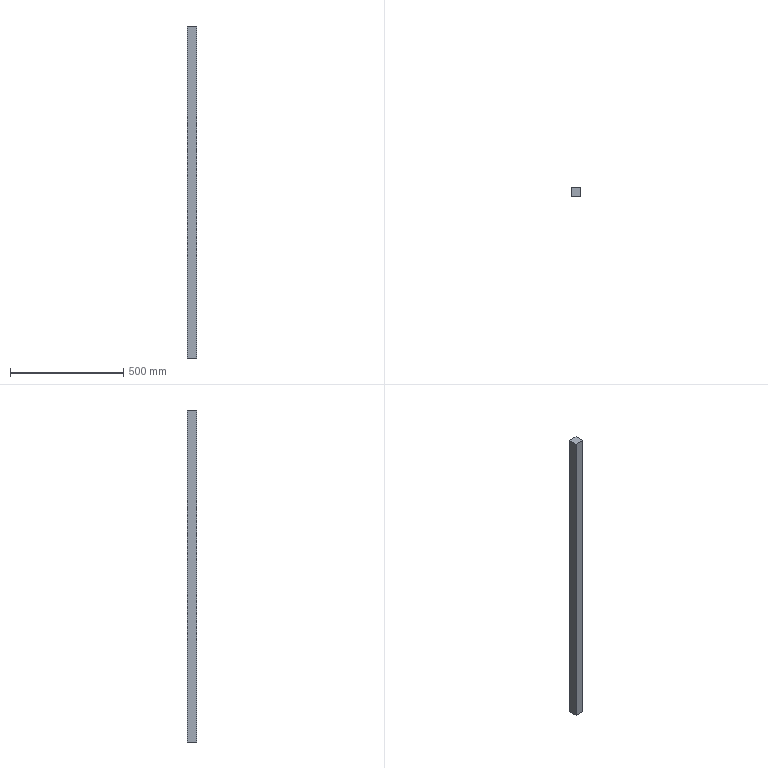Component | SolidWorks | SofaBackrest-1_SupportBar-1 | 1 solid | 6 faces | box 40 x 40 x 1468 mm | volume 2348800 mm3 | plane 6
build123d program:
from build123d import *

# Parameters (mm, degrees)
SKETCH1_W           = 40
SKETCH1_H           = 40
BOSS_EXTRUDE1_DEPTH = 1468


with BuildPart() as part:
    # Sketch1 → Boss-Extrude1 (new body)
    with BuildSketch(Plane.XY):
        with Locations((-12.665, -1.306)):
            Rectangle(SKETCH1_W, SKETCH1_H)
    extrude(amount=BOSS_EXTRUDE1_DEPTH)


solid = part.part

# Placed as in the assembly
solid = solid.moved(Location((310.484, 76.908, 846), (0, 0, 0)))
STEP:
#1=COLOUR_RGB('',0.7922,0.8196,0.9333);
#2=FILL_AREA_STYLE_COLOUR('',#1);
#3=FILL_AREA_STYLE('',(#2));
#4=SURFACE_STYLE_FILL_AREA(#3);
#5=SURFACE_SIDE_STYLE('',(#4));
#6=SURFACE_STYLE_USAGE(.BOTH.,#5);
#7=PRESENTATION_STYLE_ASSIGNMENT((#6));
#8=CARTESIAN_POINT('',(10.938,3.764,33.307));
#9=VERTEX_POINT('',#8);
#10=CARTESIAN_POINT('',(10.938,2.189,33.307));
#11=VERTEX_POINT('',#10);
#12=CARTESIAN_POINT('',(10.938,3.764,33.307));
#13=DIRECTION('',(0.,-1.,0.));
#14=VECTOR('',#13,39.37);
#15=LINE('',#12,#14);
#16=EDGE_CURVE('',#9,#11,#15,.T.);
#17=ORIENTED_EDGE('',*,*,#16,.T.);
#18=CARTESIAN_POINT('',(10.938,2.189,91.102));
#19=VERTEX_POINT('',#18);
#20=CARTESIAN_POINT('',(10.938,2.189,91.102));
#21=DIRECTION('',(0.,0.,-1.));
#22=VECTOR('',#21,39.37);
#23=LINE('',#20,#22);
#24=EDGE_CURVE('',#19,#11,#23,.T.);
#25=ORIENTED_EDGE('',*,*,#24,.F.);
#26=CARTESIAN_POINT('',(10.938,3.764,91.102));
#27=VERTEX_POINT('',#26);
#28=CARTESIAN_POINT('',(10.938,3.764,91.102));
#29=DIRECTION('',(0.,-1.,0.));
#30=VECTOR('',#29,39.37);
#31=LINE('',#28,#30);
#32=EDGE_CURVE('',#27,#19,#31,.T.);
#33=ORIENTED_EDGE('',*,*,#32,.F.);
#34=CARTESIAN_POINT('',(10.938,3.764,91.102));
#35=DIRECTION('',(0.,0.,-1.));
#36=VECTOR('',#35,39.37);
#37=LINE('',#34,#36);
#38=EDGE_CURVE('',#27,#9,#37,.T.);
#39=ORIENTED_EDGE('',*,*,#38,.T.);
#40=EDGE_LOOP('',(#17,#25,#33,#39));
#41=FACE_OUTER_BOUND('',#40,.T.);
#42=CARTESIAN_POINT('',(10.938,3.764,91.102));
#43=DIRECTION('',(1.,0.,0.));
#44=DIRECTION('',(-0.,1.,0.));
#45=AXIS2_PLACEMENT_3D('',#42,#43,#44);
#46=PLANE('',#45);
#47=ADVANCED_FACE('',(#41),#46,.F.);
#48=CARTESIAN_POINT('',(12.513,2.189,33.307));
#49=VERTEX_POINT('',#48);
#50=CARTESIAN_POINT('',(10.938,2.189,33.307));
#51=DIRECTION('',(1.,0.,0.));
#52=VECTOR('',#51,39.37);
#53=LINE('',#50,#52);
#54=EDGE_CURVE('',#11,#49,#53,.T.);
#55=ORIENTED_EDGE('',*,*,#54,.T.);
#56=CARTESIAN_POINT('',(12.513,2.189,91.102));
#57=VERTEX_POINT('',#56);
#58=CARTESIAN_POINT('',(12.513,2.189,91.102));
#59=DIRECTION('',(0.,0.,-1.));
#60=VECTOR('',#59,39.37);
#61=LINE('',#58,#60);
#62=EDGE_CURVE('',#57,#49,#61,.T.);
#63=ORIENTED_EDGE('',*,*,#62,.F.);
#64=CARTESIAN_POINT('',(10.938,2.189,91.102));
#65=DIRECTION('',(1.,0.,0.));
#66=VECTOR('',#65,39.37);
#67=LINE('',#64,#66);
#68=EDGE_CURVE('',#19,#57,#67,.T.);
#69=ORIENTED_EDGE('',*,*,#68,.F.);
#70=ORIENTED_EDGE('',*,*,#24,.T.);
#71=EDGE_LOOP('',(#55,#63,#69,#70));
#72=FACE_OUTER_BOUND('',#71,.T.);
#73=CARTESIAN_POINT('',(10.938,2.189,91.102));
#74=DIRECTION('',(0.,1.,0.));
#75=DIRECTION('',(0.,0.,1.));
#76=AXIS2_PLACEMENT_3D('',#73,#74,#75);
#77=PLANE('',#76);
#78=ADVANCED_FACE('',(#72),#77,.F.);
#79=CARTESIAN_POINT('',(12.513,3.764,33.307));
#80=VERTEX_POINT('',#79);
#81=CARTESIAN_POINT('',(12.513,3.764,33.307));
#82=DIRECTION('',(-0.,1.,0.));
#83=VECTOR('',#82,39.37);
#84=LINE('',#81,#83);
#85=EDGE_CURVE('',#49,#80,#84,.T.);
#86=ORIENTED_EDGE('',*,*,#85,.T.);
#87=CARTESIAN_POINT('',(12.513,3.764,91.102));
#88=VERTEX_POINT('',#87);
#89=CARTESIAN_POINT('',(12.513,3.764,91.102));
#90=DIRECTION('',(0.,0.,-1.));
#91=VECTOR('',#90,39.37);
#92=LINE('',#89,#91);
#93=EDGE_CURVE('',#88,#80,#92,.T.);
#94=ORIENTED_EDGE('',*,*,#93,.F.);
#95=CARTESIAN_POINT('',(12.513,3.764,91.102));
#96=DIRECTION('',(-0.,1.,0.));
#97=VECTOR('',#96,39.37);
#98=LINE('',#95,#97);
#99=EDGE_CURVE('',#57,#88,#98,.T.);
#100=ORIENTED_EDGE('',*,*,#99,.F.);
#101=ORIENTED_EDGE('',*,*,#62,.T.);
#102=EDGE_LOOP('',(#86,#94,#100,#101));
#103=FACE_OUTER_BOUND('',#102,.T.);
#104=CARTESIAN_POINT('',(12.513,3.764,91.102));
#105=DIRECTION('',(-1.,-0.,0.));
#106=DIRECTION('',(0.,-1.,0.));
#107=AXIS2_PLACEMENT_3D('',#104,#105,#106);
#108=PLANE('',#107);
#109=ADVANCED_FACE('',(#103),#108,.F.);
#110=CARTESIAN_POINT('',(10.938,3.764,33.307));
#111=DIRECTION('',(-1.,0.,0.));
#112=VECTOR('',#111,39.37);
#113=LINE('',#110,#112);
#114=EDGE_CURVE('',#80,#9,#113,.T.);
#115=ORIENTED_EDGE('',*,*,#114,.T.);
#116=ORIENTED_EDGE('',*,*,#38,.F.);
#117=CARTESIAN_POINT('',(10.938,3.764,91.102));
#118=DIRECTION('',(-1.,0.,0.));
#119=VECTOR('',#118,39.37);
#120=LINE('',#117,#119);
#121=EDGE_CURVE('',#88,#27,#120,.T.);
#122=ORIENTED_EDGE('',*,*,#121,.F.);
#123=ORIENTED_EDGE('',*,*,#93,.T.);
#124=EDGE_LOOP('',(#115,#116,#122,#123));
#125=FACE_OUTER_BOUND('',#124,.T.);
#126=CARTESIAN_POINT('',(10.938,3.764,91.102));
#127=DIRECTION('',(0.,-1.,0.));
#128=DIRECTION('',(0.,0.,-1.));
#129=AXIS2_PLACEMENT_3D('',#126,#127,#128);
#130=PLANE('',#129);
#131=ADVANCED_FACE('',(#125),#130,.F.);
#132=ORIENTED_EDGE('',*,*,#32,.T.);
#133=ORIENTED_EDGE('',*,*,#68,.T.);
#134=ORIENTED_EDGE('',*,*,#99,.T.);
#135=ORIENTED_EDGE('',*,*,#121,.T.);
#136=EDGE_LOOP('',(#132,#133,#134,#135));
#137=FACE_OUTER_BOUND('',#136,.T.);
#138=CARTESIAN_POINT('',(12.224,3.028,91.102));
#139=DIRECTION('',(0.,0.,1.));
#140=DIRECTION('',(1.,0.,0.));
#141=AXIS2_PLACEMENT_3D('',#138,#139,#140);
#142=PLANE('',#141);
#143=ADVANCED_FACE('',(#137),#142,.T.);
#144=ORIENTED_EDGE('',*,*,#16,.F.);
#145=ORIENTED_EDGE('',*,*,#114,.F.);
#146=ORIENTED_EDGE('',*,*,#85,.F.);
#147=ORIENTED_EDGE('',*,*,#54,.F.);
#148=EDGE_LOOP('',(#144,#145,#146,#147));
#149=FACE_OUTER_BOUND('',#148,.T.);
#150=CARTESIAN_POINT('',(12.224,3.028,33.307));
#151=DIRECTION('',(0.,0.,1.));
#152=DIRECTION('',(1.,0.,0.));
#153=AXIS2_PLACEMENT_3D('',#150,#151,#152);
#154=PLANE('',#153);
#155=ADVANCED_FACE('',(#149),#154,.F.);
#156=CLOSED_SHELL('',(#47,#78,#109,#131,#143,#155));
#157=MANIFOLD_SOLID_BREP('',#156);
#158=STYLED_ITEM('',(#7),#157);
#159=(LENGTH_UNIT()NAMED_UNIT(*)SI_UNIT($,.METRE.));
#160=LENGTH_MEASURE_WITH_UNIT(LENGTH_MEASURE(0.0254),#159);
#161=DIMENSIONAL_EXPONENTS(1.,0.,0.,0.,0.,0.,0.);
#162=(CONVERSION_BASED_UNIT('',#160)LENGTH_UNIT()NAMED_UNIT(#161));
#163=UNCERTAINTY_MEASURE_WITH_UNIT(LENGTH_MEASURE(0.00001),#162,'','');
#164=(NAMED_UNIT(*)PLANE_ANGLE_UNIT()SI_UNIT($,.RADIAN.));
#165=(NAMED_UNIT(*)SI_UNIT($,.STERADIAN.)SOLID_ANGLE_UNIT());
#166=(GEOMETRIC_REPRESENTATION_CONTEXT(3)GLOBAL_UNCERTAINTY_ASSIGNED_CONTEXT((#163))GLOBAL_UNIT_ASSIGNED_CONTEXT((#162,#164,#165))REPRESENTATION_CONTEXT('',''));
#167=MECHANICAL_DESIGN_GEOMETRIC_PRESENTATION_REPRESENTATION('',(#158),#166);
#168=PRESENTATION_LAYER_ASSIGNMENT('','',(#158));
#169=CARTESIAN_POINT('',(0.,0.,0.));
#170=DIRECTION('',(0.,0.,1.));
#171=DIRECTION('',(1.,0.,0.));
#172=AXIS2_PLACEMENT_3D('',#169,#170,#171);
#173=(LENGTH_UNIT()NAMED_UNIT(*)SI_UNIT($,.METRE.));
#174=LENGTH_MEASURE_WITH_UNIT(LENGTH_MEASURE(0.0254),#173);
#175=DIMENSIONAL_EXPONENTS(1.,0.,0.,0.,0.,0.,0.);
#176=(CONVERSION_BASED_UNIT('',#174)LENGTH_UNIT()NAMED_UNIT(#175));
#177=UNCERTAINTY_MEASURE_WITH_UNIT(LENGTH_MEASURE(0.00001),#176,'','');
#178=(NAMED_UNIT(*)PLANE_ANGLE_UNIT()SI_UNIT($,.RADIAN.));
#179=(NAMED_UNIT(*)SI_UNIT($,.STERADIAN.)SOLID_ANGLE_UNIT());
#180=(GEOMETRIC_REPRESENTATION_CONTEXT(3)GLOBAL_UNCERTAINTY_ASSIGNED_CONTEXT((#177))GLOBAL_UNIT_ASSIGNED_CONTEXT((#176,#178,#179))REPRESENTATION_CONTEXT('',''));
#181=ADVANCED_BREP_SHAPE_REPRESENTATION('',(#157,#172),#180);